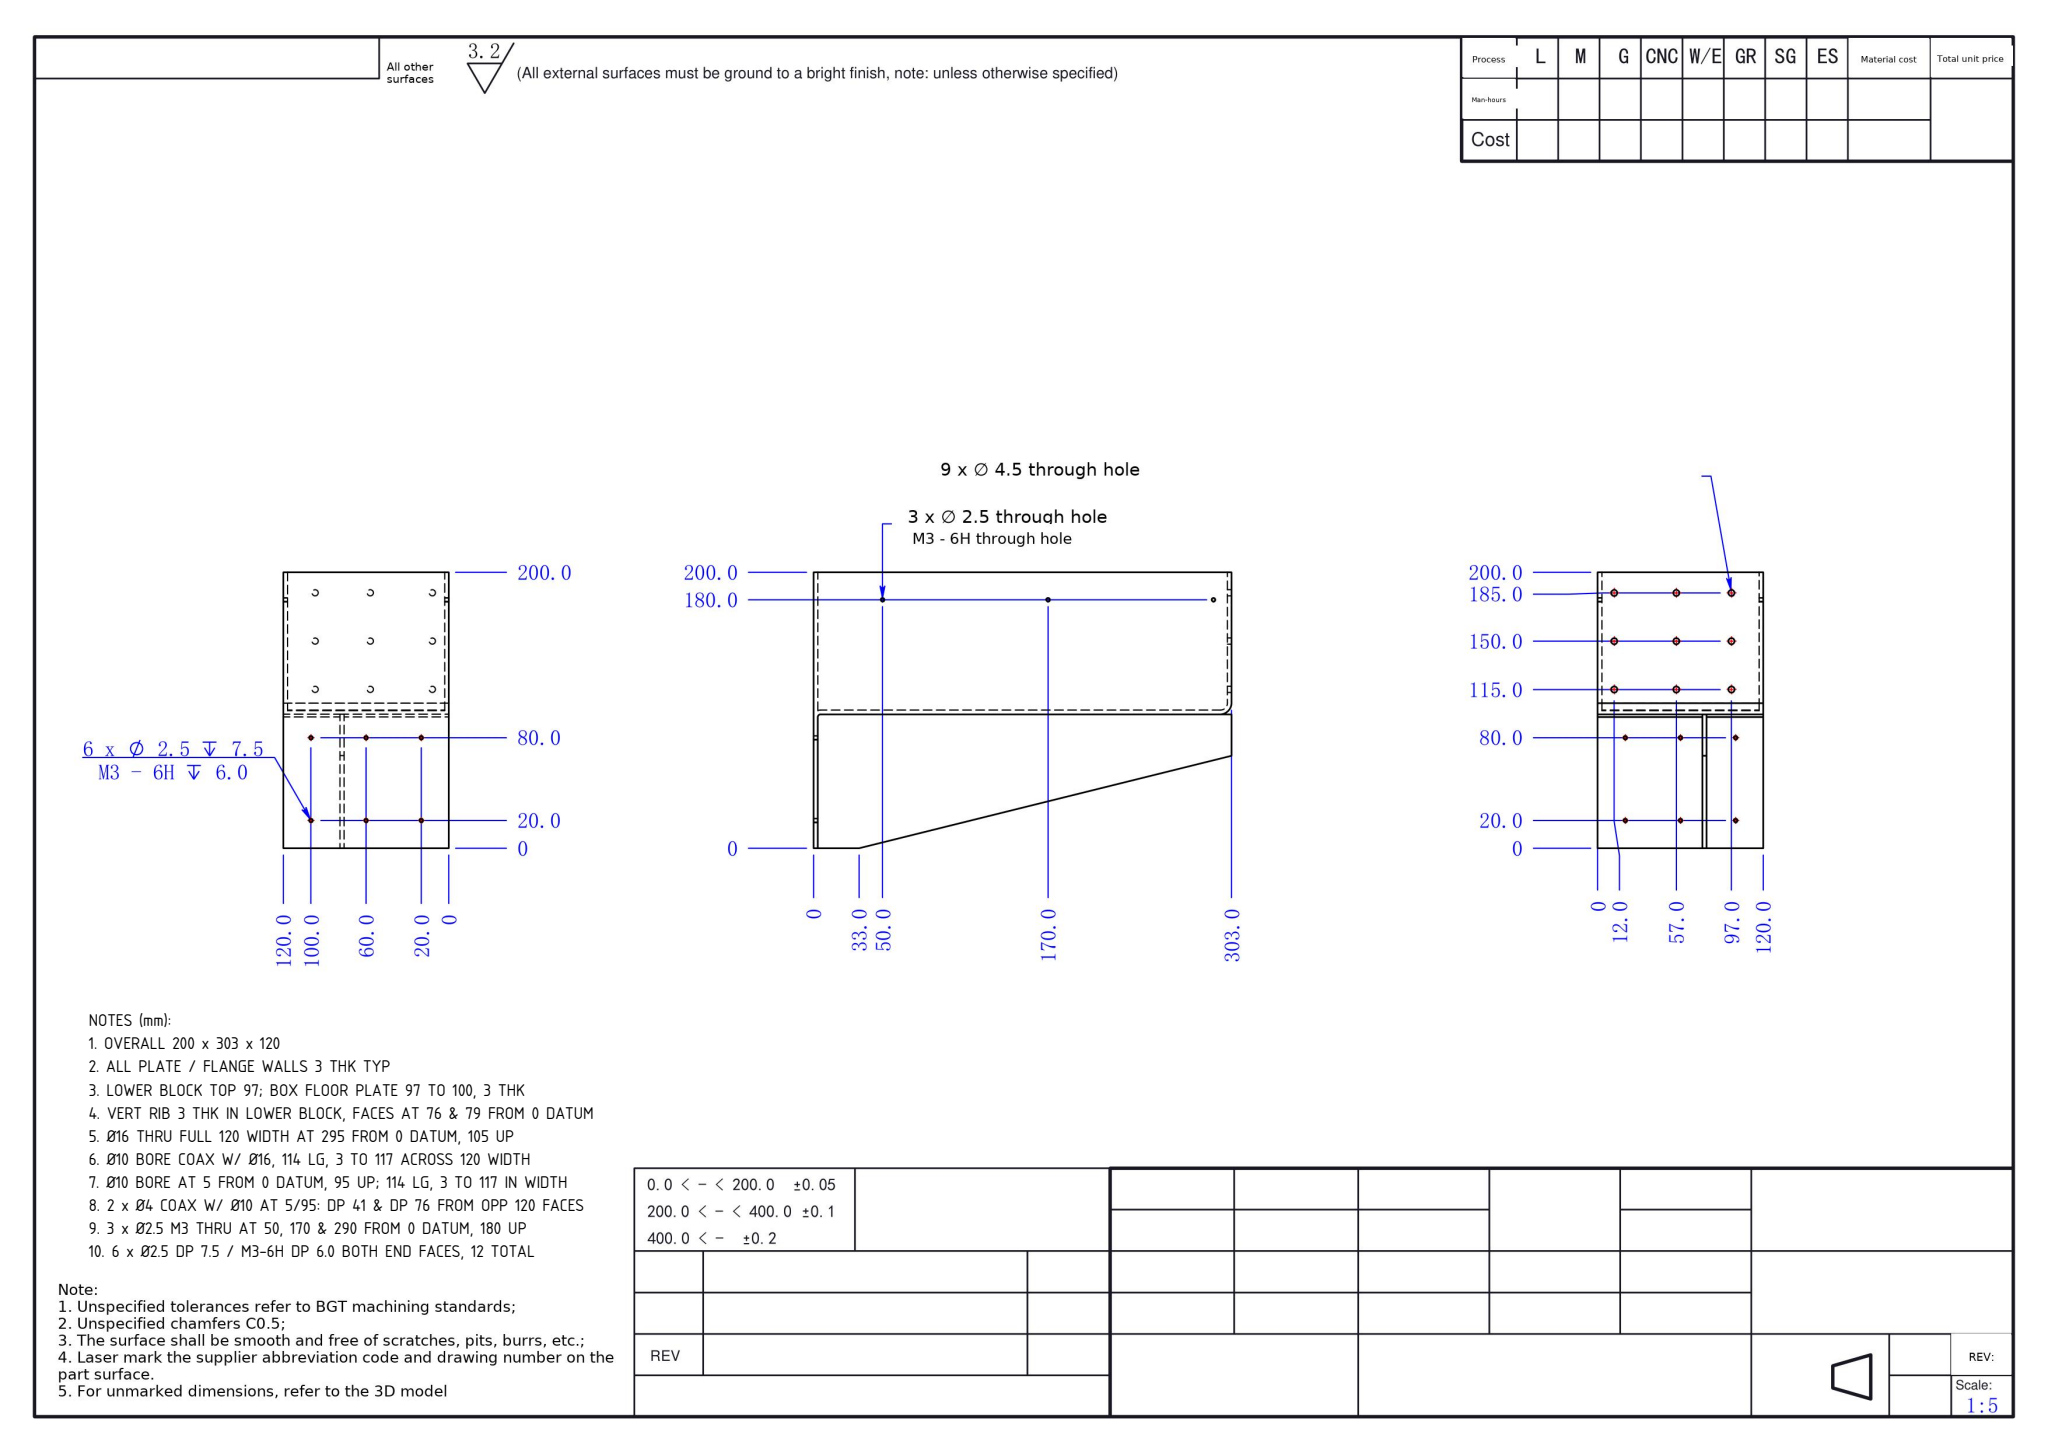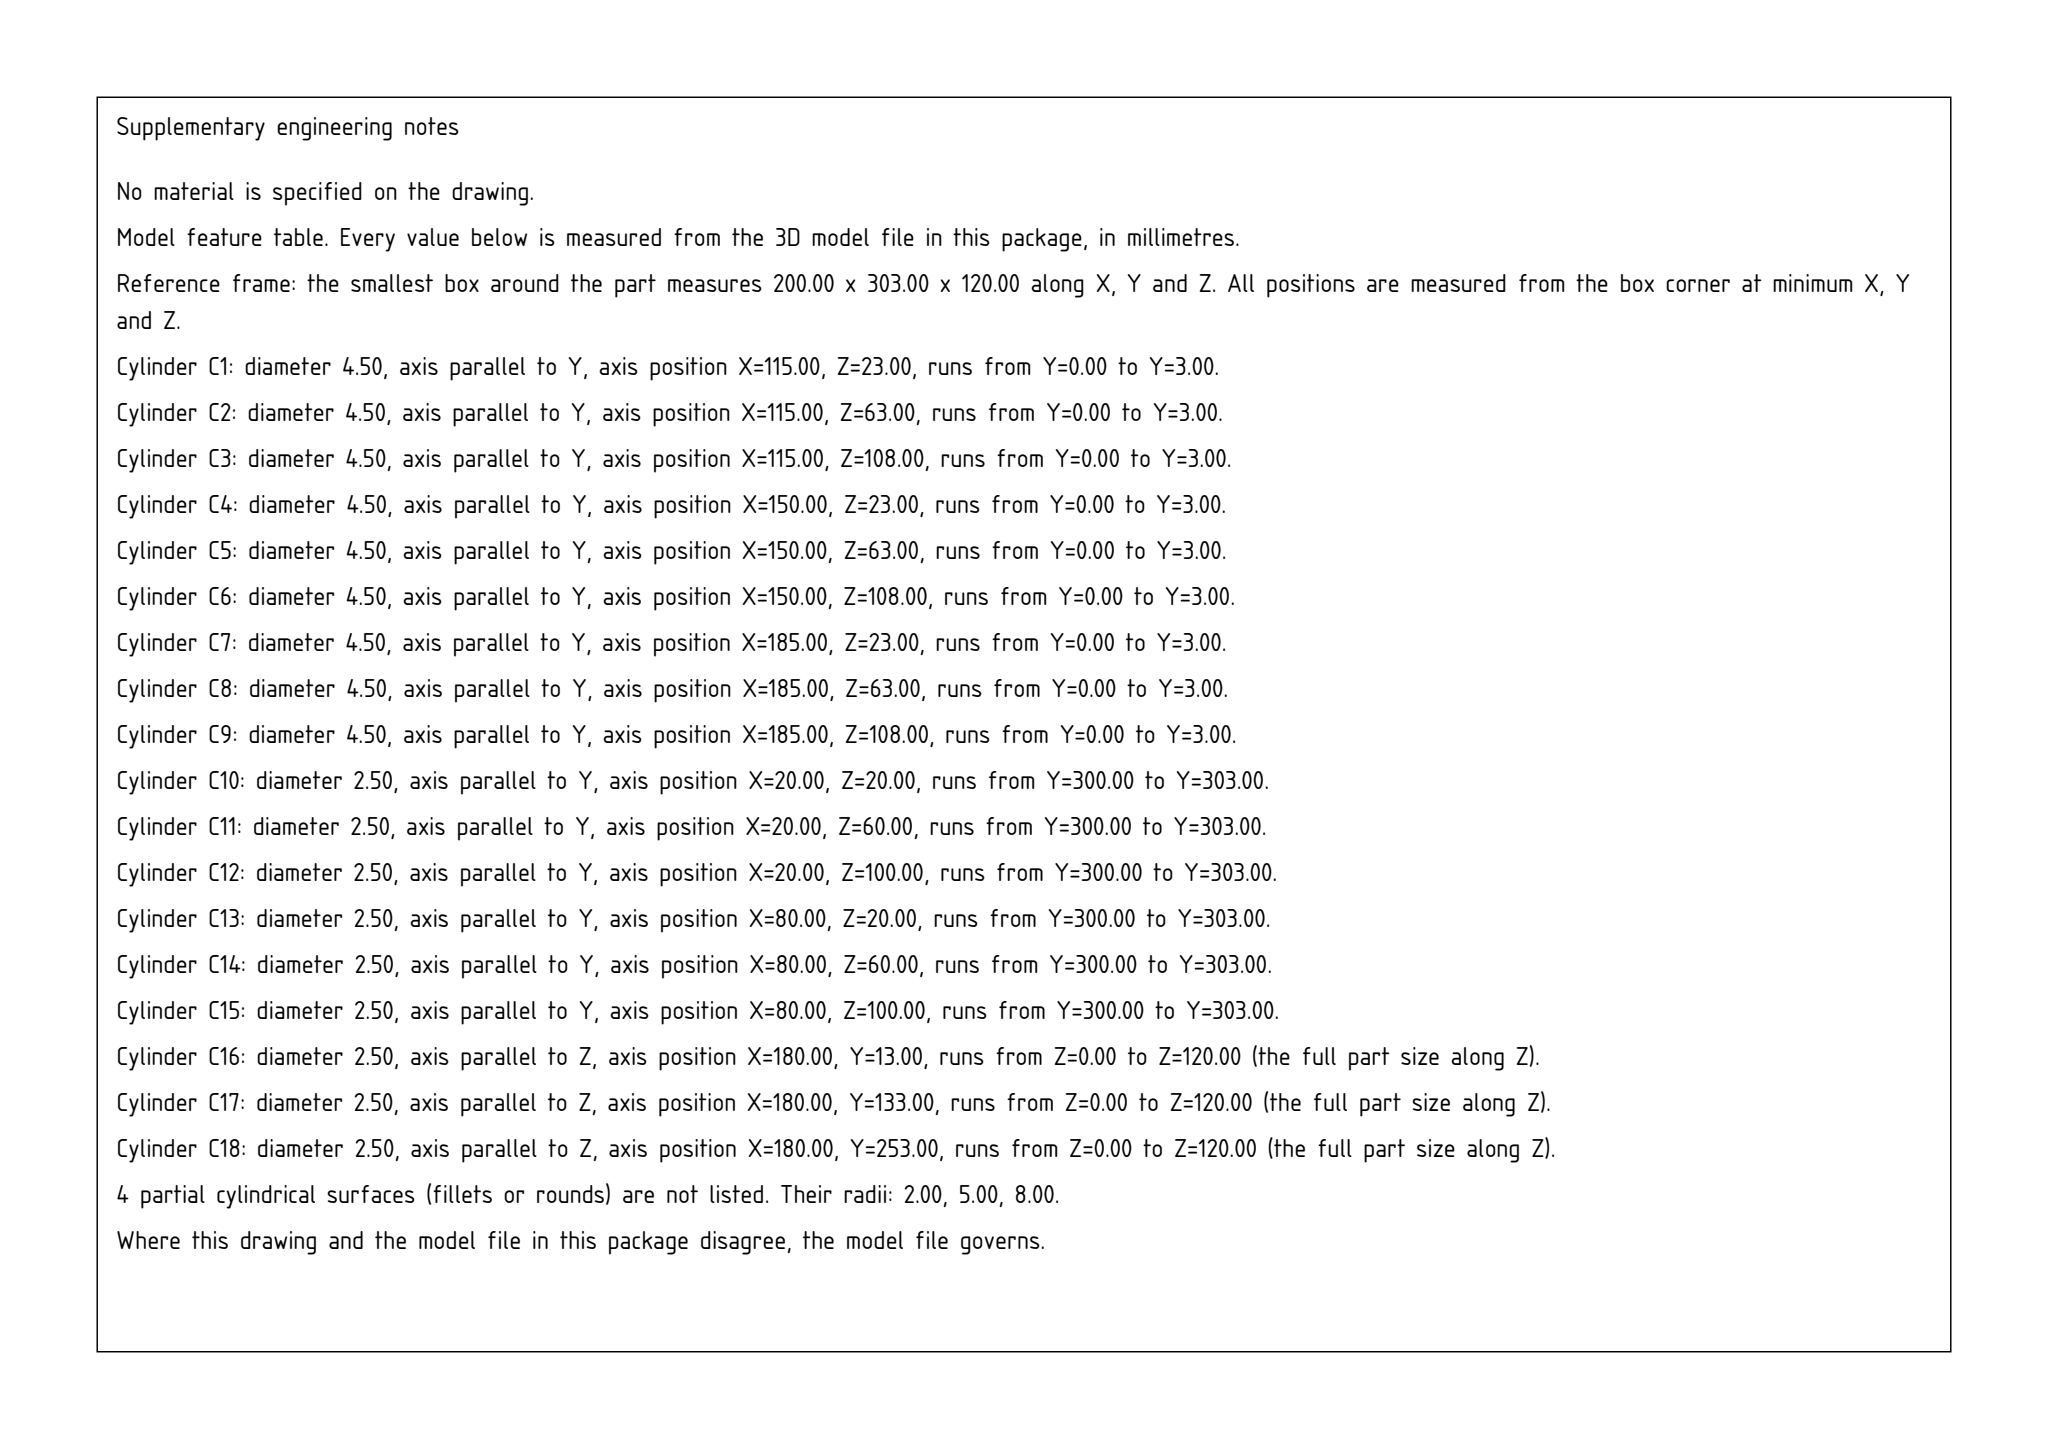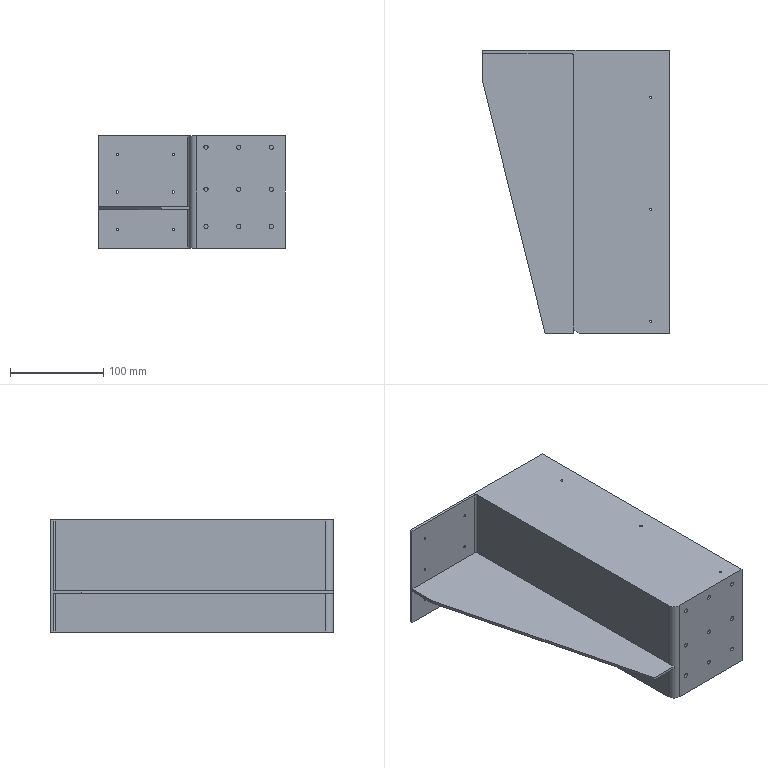Part | SolidWorks | mm | 1 solid | 67 faces | box 200 x 303 x 120 mm | volume 452792 mm3 | cylinder 47 | plane 20 | commonest cylinder face diameters 2.5 x24 4.5 x18 10 x2 4 x2 16 x1
Drawing notes:
OVERALL 200 x 303 x 120 | from the solid: bbox_xyz = [200.0, 303.0, 120.0]
ALL PLATE / FLANGE WALLS 3 THK TYP | from the solid: planes y=0/3 & y=300/303, z=0/3 & z=117/120, x=97/100 -> 3 mm skins
LOWER BLOCK TOP 97; BOX FLOOR PLATE 97 TO 100, 3 THK | from the solid: x-normal planes 0, 97 (x3), 100, 200; upper box 100-200, lower block 0-97
VERT RIB 3 THK IN LOWER BLOCK, FACES AT 76 & 79 FROM 0 DATUM | from the solid: z-normal planes 41 & 44 = 76 & 79 from z=120 face (right-view 0 datum)
Ø16 THRU FULL 120 WIDTH AT 295 FROM 0 DATUM, 105 UP | from the solid: cyl dia16 axis z pos(x=105,y=8) len120; 303-8=295 from LH end face
Ø10 BORE COAX W/ Ø16, 114 LG, 3 TO 117 ACROSS 120 WIDTH | from the solid: cyl dia10 axis z pos(105,8) len114; z planes 3 & 117 (117-3=114)
Ø10 BORE AT 5 FROM 0 DATUM, 95 UP; 114 LG, 3 TO 117 IN WIDTH | from the solid: cyl dia10 axis z pos(x=95,y=298) len114; 303-298=5; z planes 3/117
2 x Ø4 COAX W/ Ø10 AT 5/95: DP 41 & DP 76 FROM OPP 120 FACES | from the solid: cyl dia4 axis z pos(95,298) len41 & len76; z planes 41 & 44; 44+76=120
3 x Ø2.5 M3 THRU AT 50, 170 & 290 FROM 0 DATUM, 180 UP | from the solid: dia2.5 axis z at x=180, y=13/133/253; 303-13=290, -133=170, -253=50
6 x Ø2.5 DP 7.5 / M3-6H DP 6.0 BOTH END FACES, 12 TOTAL | from the solid: each dia2.5 axis y hole count=2 (y=0-3 and y=300-303 end plates)
build123d program:
from build123d import *

# Parameters (mm, degrees)
EXTRUDE_THIN1_DEPTH            = 120
BOSS_EXTRUDE1_DEPTH            = 1.5
BOSS_EXTRUDE2_START            = -3
BOSS_EXTRUDE2_DEPTH            = 3
BOSS_EXTRUDE3_DEPTH            = 3
SKETCH5_W                      = 120
SKETCH5_H                      = 3
BOSS_EXTRUDE4_DEPTH            = 200
F_4_5_4_5_DIAMETER_HOLE1_D     = 4.5
F_4_5_4_5_DIAMETER_HOLE1_DEPTH = 3
M3_TAPPED_HOLE1_D              = 2.5
M3_TAPPED_HOLE1_DEPTH          = 7.5
M3_TAPPED_HOLE1_TIP            = 0.7511
M3_TAPPED_HOLE2_D              = 2.5


with BuildPart() as part:
    # Sketch1 → Extrude-Thin1 (new body)
    with BuildSketch(Plane.XY):
        with BuildLine():
            Line((0, 0), (95, 0))
            ThreePointArc((95, 0), (98.536, -1.464), (100, -5))
            Line((100, -5), (100, -295))
            ThreePointArc((100, -295), (101.464, -298.536), (105, -300))
            Line((105, -300), (200, -300))
            Line((200, -300), (200, -303))
            Line((200, -303), (105, -303))
            ThreePointArc((105, -303), (99.343, -300.657), (97, -295))
            Line((97, -295), (97, -5))
            ThreePointArc((97, -5), (96.414, -3.586), (95, -3))
            Line((95, -3), (0, -3))
            Line((0, -3), (0, 0))
        make_face()
    extrude(amount=EXTRUDE_THIN1_DEPTH)

    # Sketch2 → Boss-Extrude1 (add, symmetric)
    with BuildSketch(Plane.XY.offset(42.5)):
        with BuildLine():
            Line((0, -3), (95, -3))
            ThreePointArc((95, -3), (96.414, -3.586), (97, -5))
            Line((97, -5), (97, -303))
            Line((97, -303), (67, -303))
            Line((67, -303), (0, -33))
            Line((0, -33), (0, -3))
        make_face()
    extrude(amount=BOSS_EXTRUDE1_DEPTH, both=True)

    # Sketch3 → Boss-Extrude2 (add)
    with BuildSketch(Plane.XY.offset(120).offset(BOSS_EXTRUDE2_START)):
        with BuildLine():
            Line((200, -303), (200, 0))
            Line((200, 0), (97, 0))
            Line((97, 0), (97, -295))
            ThreePointArc((97, -295), (99.343, -300.657), (105, -303))
            Line((105, -303), (200, -303))
        make_face()
    extrude(amount=BOSS_EXTRUDE2_DEPTH)

    # Sketch4 → Boss-Extrude3 (add)
    with BuildSketch(Plane(origin=(0, 0, 0), x_dir=(-1, 0, 0), z_dir=(0, 0, -1))):
        with BuildLine():
            Line((-97, 0), (-200, 0))
            Line((-200, 0), (-200, -303))
            Line((-200, -303), (-105, -303))
            ThreePointArc((-105, -303), (-99.343, -300.657), (-97, -295))
            Line((-97, -295), (-97, 0))
        make_face()
    extrude(amount=-BOSS_EXTRUDE3_DEPTH)

    # Sketch5 → Boss-Extrude4 (add)
    with BuildSketch(Plane.ZY):
        with Locations((60, -1.5)):
            Rectangle(SKETCH5_W, SKETCH5_H)
    extrude(amount=-BOSS_EXTRUDE4_DEPTH)

    # 4.5 _4.5_ Diameter Hole1
    with Locations(Plane(origin=(0, -300, 0), x_dir=(1, 0, 0), z_dir=(0, 1, 0))):
        with Locations((115, -23), (150, -23), (185, -23), (115, -108), (150, -108), (185, -108), (115, -63), (150, -63), (185, -63)):
            Hole(F_4_5_4_5_DIAMETER_HOLE1_D / 2, depth=F_4_5_4_5_DIAMETER_HOLE1_DEPTH)

    # M3 Tapped Hole1
    with Locations(Plane(origin=(0, 0, 0), x_dir=(1, 0, 0), z_dir=(0, 1, 0))):
        with Locations((80, -20), (80, -60), (80, -100), (20, -100), (20, -60), (20, -20)):
            Hole(M3_TAPPED_HOLE1_D / 2, depth=M3_TAPPED_HOLE1_DEPTH)
            with Locations((0, 0, -(M3_TAPPED_HOLE1_DEPTH + M3_TAPPED_HOLE1_TIP / 2))):  # 118° drill point
                Cone(0, M3_TAPPED_HOLE1_D / 2, M3_TAPPED_HOLE1_TIP, mode=Mode.SUBTRACT)

    # M3 Tapped Hole2 (through all)
    with Locations(Plane.XY.offset(120)):
        with Locations((180, -50), (180, -170), (180, -290)):
            Hole(M3_TAPPED_HOLE2_D / 2)


solid = part.part